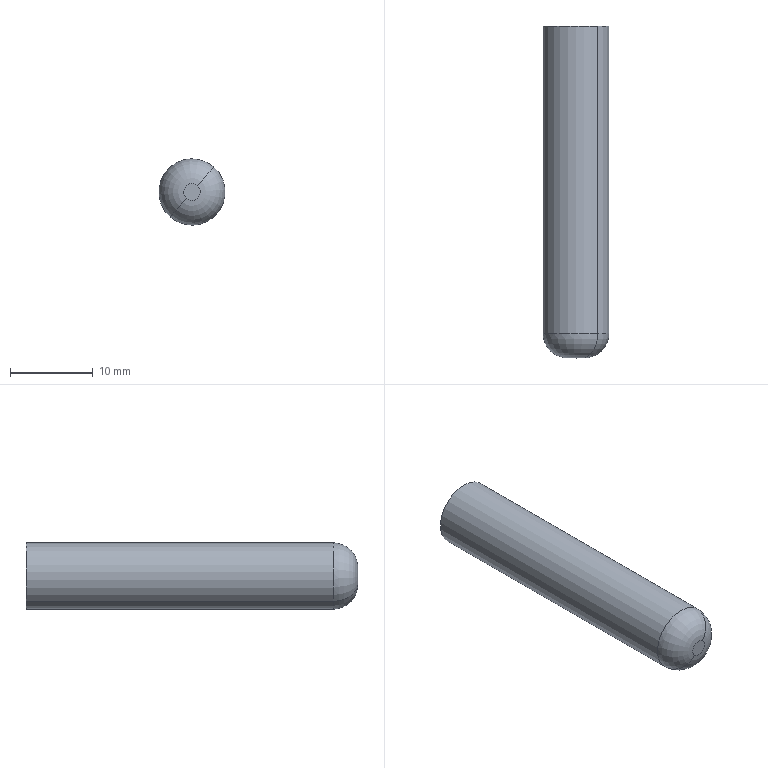Component | SolidWorks | NewDieSet-1_LocatingPin-1 | 1 solid | 6 faces | box 8 x 40 x 8 mm | volume 1970 mm3 | torus 2 | cylinder 2 | plane 2 | commonest cylinder face diameters 8 x2
build123d program:
from build123d import *

# Parameters (mm, degrees)
SKETCH1_R           = 4
BOSS_EXTRUDE1_DEPTH = 40
FILLET1_R           = 3


with BuildPart() as part:
    # Sketch1 → Boss-Extrude1 (new body)
    with BuildSketch(Plane.XY):
        Circle(SKETCH1_R)
    extrude(amount=BOSS_EXTRUDE1_DEPTH)

    # Fillet1
    fillet1_edges = [part.edges().sort_by_distance(p)[0] for p in [
        (-4, 0, 0),
    ]]
    fillet(fillet1_edges, radius=FILLET1_R)


solid = part.part

# Placed as in the assembly
solid = solid.moved(Location((-146.746, -9.073, 551.1), (-90, 0, 0)))
STEP:
#1=CARTESIAN_POINT('',(-5.803,-0.3572,21.667));
#2=VERTEX_POINT('',#1);
#3=CARTESIAN_POINT('',(-5.752,-0.3572,21.727));
#4=VERTEX_POINT('',#3);
#5=CARTESIAN_POINT('',(-5.777,-0.3572,21.697));
#6=DIRECTION('',(-0.,-1.,0.));
#7=DIRECTION('',(0.6544,0.,0.7562));
#8=AXIS2_PLACEMENT_3D('',#5,#6,#7);
#9=CIRCLE('',#8,0.03937);
#10=EDGE_CURVE('',#2,#4,#9,.T.);
#11=ORIENTED_EDGE('',*,*,#10,.F.);
#12=CARTESIAN_POINT('',(-5.88,-0.2391,21.578));
#13=VERTEX_POINT('',#12);
#14=CARTESIAN_POINT('',(-5.803,-0.2391,21.667));
#15=DIRECTION('',(0.7562,-0.,-0.6544));
#16=DIRECTION('',(-0.6544,0.,-0.7562));
#17=AXIS2_PLACEMENT_3D('',#14,#15,#16);
#18=CIRCLE('',#17,0.1181);
#19=EDGE_CURVE('',#2,#13,#18,.T.);
#20=ORIENTED_EDGE('',*,*,#19,.T.);
#21=CARTESIAN_POINT('',(-5.674,-0.2391,21.816));
#22=VERTEX_POINT('',#21);
#23=CARTESIAN_POINT('',(-5.777,-0.2391,21.697));
#24=DIRECTION('',(0.,1.,-0.));
#25=DIRECTION('',(0.6544,0.,0.7562));
#26=AXIS2_PLACEMENT_3D('',#23,#24,#25);
#27=CIRCLE('',#26,0.1575);
#28=EDGE_CURVE('',#22,#13,#27,.T.);
#29=ORIENTED_EDGE('',*,*,#28,.F.);
#30=CARTESIAN_POINT('',(-5.752,-0.2391,21.727));
#31=DIRECTION('',(-0.7562,0.,0.6544));
#32=DIRECTION('',(0.6544,0.,0.7562));
#33=AXIS2_PLACEMENT_3D('',#30,#31,#32);
#34=CIRCLE('',#33,0.1181);
#35=EDGE_CURVE('',#4,#22,#34,.T.);
#36=ORIENTED_EDGE('',*,*,#35,.F.);
#37=EDGE_LOOP('',(#11,#20,#29,#36));
#38=FACE_OUTER_BOUND('',#37,.T.);
#39=CARTESIAN_POINT('',(-5.777,-0.2391,21.697));
#40=DIRECTION('',(0.,1.,-0.));
#41=DIRECTION('',(0.6544,-0.,0.7562));
#42=AXIS2_PLACEMENT_3D('',#39,#40,#41);
#43=TOROIDAL_SURFACE('',#42,0.03937,0.1181);
#44=ADVANCED_FACE('',(#38),#43,.T.);
#45=CARTESIAN_POINT('',(-5.674,1.218,21.816));
#46=VERTEX_POINT('',#45);
#47=CARTESIAN_POINT('',(-5.88,1.218,21.578));
#48=VERTEX_POINT('',#47);
#49=CARTESIAN_POINT('',(-5.777,1.218,21.697));
#50=DIRECTION('',(0.,1.,-0.));
#51=DIRECTION('',(0.6544,0.,0.7562));
#52=AXIS2_PLACEMENT_3D('',#49,#50,#51);
#53=CIRCLE('',#52,0.1575);
#54=EDGE_CURVE('',#46,#48,#53,.T.);
#55=ORIENTED_EDGE('',*,*,#54,.F.);
#56=CARTESIAN_POINT('',(-5.674,1.218,21.816));
#57=DIRECTION('',(-0.,-1.,0.));
#58=VECTOR('',#57,39.37);
#59=LINE('',#56,#58);
#60=EDGE_CURVE('',#46,#22,#59,.T.);
#61=ORIENTED_EDGE('',*,*,#60,.T.);
#62=ORIENTED_EDGE('',*,*,#28,.T.);
#63=CARTESIAN_POINT('',(-5.88,1.218,21.578));
#64=DIRECTION('',(-0.,-1.,0.));
#65=VECTOR('',#64,39.37);
#66=LINE('',#63,#65);
#67=EDGE_CURVE('',#48,#13,#66,.T.);
#68=ORIENTED_EDGE('',*,*,#67,.F.);
#69=EDGE_LOOP('',(#55,#61,#62,#68));
#70=FACE_OUTER_BOUND('',#69,.T.);
#71=CARTESIAN_POINT('',(-5.777,1.218,21.697));
#72=DIRECTION('',(-0.,-1.,0.));
#73=DIRECTION('',(-0.6544,0.,-0.7562));
#74=AXIS2_PLACEMENT_3D('',#71,#72,#73);
#75=CYLINDRICAL_SURFACE('',#74,0.1575);
#76=ADVANCED_FACE('',(#70),#75,.T.);
#77=ORIENTED_EDGE('',*,*,#60,.F.);
#78=CARTESIAN_POINT('',(-5.777,1.218,21.697));
#79=DIRECTION('',(0.,1.,-0.));
#80=DIRECTION('',(0.6544,0.,0.7562));
#81=AXIS2_PLACEMENT_3D('',#78,#79,#80);
#82=CIRCLE('',#81,0.1575);
#83=EDGE_CURVE('',#48,#46,#82,.T.);
#84=ORIENTED_EDGE('',*,*,#83,.F.);
#85=ORIENTED_EDGE('',*,*,#67,.T.);
#86=CARTESIAN_POINT('',(-5.777,-0.2391,21.697));
#87=DIRECTION('',(0.,1.,-0.));
#88=DIRECTION('',(0.6544,0.,0.7562));
#89=AXIS2_PLACEMENT_3D('',#86,#87,#88);
#90=CIRCLE('',#89,0.1575);
#91=EDGE_CURVE('',#13,#22,#90,.T.);
#92=ORIENTED_EDGE('',*,*,#91,.T.);
#93=EDGE_LOOP('',(#77,#84,#85,#92));
#94=FACE_OUTER_BOUND('',#93,.T.);
#95=CARTESIAN_POINT('',(-5.777,1.218,21.697));
#96=DIRECTION('',(-0.,-1.,0.));
#97=DIRECTION('',(-0.6544,0.,-0.7562));
#98=AXIS2_PLACEMENT_3D('',#95,#96,#97);
#99=CYLINDRICAL_SURFACE('',#98,0.1575);
#100=ADVANCED_FACE('',(#94),#99,.T.);
#101=ORIENTED_EDGE('',*,*,#83,.T.);
#102=ORIENTED_EDGE('',*,*,#54,.T.);
#103=EDGE_LOOP('',(#101,#102));
#104=FACE_OUTER_BOUND('',#103,.T.);
#105=CARTESIAN_POINT('',(-5.777,1.218,21.697));
#106=DIRECTION('',(0.,1.,-0.));
#107=DIRECTION('',(0.6544,-0.,0.7562));
#108=AXIS2_PLACEMENT_3D('',#105,#106,#107);
#109=PLANE('',#108);
#110=ADVANCED_FACE('',(#104),#109,.T.);
#111=CARTESIAN_POINT('',(-5.777,-0.3572,21.697));
#112=DIRECTION('',(-0.,-1.,0.));
#113=DIRECTION('',(0.6544,0.,0.7562));
#114=AXIS2_PLACEMENT_3D('',#111,#112,#113);
#115=CIRCLE('',#114,0.03937);
#116=EDGE_CURVE('',#4,#2,#115,.T.);
#117=ORIENTED_EDGE('',*,*,#116,.T.);
#118=ORIENTED_EDGE('',*,*,#10,.T.);
#119=EDGE_LOOP('',(#117,#118));
#120=FACE_OUTER_BOUND('',#119,.T.);
#121=CARTESIAN_POINT('',(-5.777,-0.3572,21.697));
#122=DIRECTION('',(0.,1.,-0.));
#123=DIRECTION('',(0.6544,-0.,0.7562));
#124=AXIS2_PLACEMENT_3D('',#121,#122,#123);
#125=PLANE('',#124);
#126=ADVANCED_FACE('',(#120),#125,.F.);
#127=ORIENTED_EDGE('',*,*,#19,.F.);
#128=ORIENTED_EDGE('',*,*,#116,.F.);
#129=ORIENTED_EDGE('',*,*,#35,.T.);
#130=ORIENTED_EDGE('',*,*,#91,.F.);
#131=EDGE_LOOP('',(#127,#128,#129,#130));
#132=FACE_OUTER_BOUND('',#131,.T.);
#133=CARTESIAN_POINT('',(-5.777,-0.2391,21.697));
#134=DIRECTION('',(0.,1.,-0.));
#135=DIRECTION('',(0.6544,-0.,0.7562));
#136=AXIS2_PLACEMENT_3D('',#133,#134,#135);
#137=TOROIDAL_SURFACE('',#136,0.03937,0.1181);
#138=ADVANCED_FACE('',(#132),#137,.T.);
#139=CLOSED_SHELL('',(#44,#76,#100,#110,#126,#138));
#140=MANIFOLD_SOLID_BREP('',#139);
#141=CARTESIAN_POINT('',(0.,0.,0.));
#142=DIRECTION('',(0.,0.,1.));
#143=DIRECTION('',(1.,0.,0.));
#144=AXIS2_PLACEMENT_3D('',#141,#142,#143);
#145=(LENGTH_UNIT()NAMED_UNIT(*)SI_UNIT($,.METRE.));
#146=LENGTH_MEASURE_WITH_UNIT(LENGTH_MEASURE(0.0254),#145);
#147=DIMENSIONAL_EXPONENTS(1.,0.,0.,0.,0.,0.,0.);
#148=(CONVERSION_BASED_UNIT('',#146)LENGTH_UNIT()NAMED_UNIT(#147));
#149=UNCERTAINTY_MEASURE_WITH_UNIT(LENGTH_MEASURE(0.00001),#148,'','');
#150=(NAMED_UNIT(*)PLANE_ANGLE_UNIT()SI_UNIT($,.RADIAN.));
#151=(NAMED_UNIT(*)SI_UNIT($,.STERADIAN.)SOLID_ANGLE_UNIT());
#152=(GEOMETRIC_REPRESENTATION_CONTEXT(3)GLOBAL_UNCERTAINTY_ASSIGNED_CONTEXT((#149))GLOBAL_UNIT_ASSIGNED_CONTEXT((#148,#150,#151))REPRESENTATION_CONTEXT('',''));
#153=ADVANCED_BREP_SHAPE_REPRESENTATION('',(#140,#144),#152);
#154=COLOUR_RGB('',0.7922,0.8196,0.9333);
#155=FILL_AREA_STYLE_COLOUR('',#154);
#156=FILL_AREA_STYLE('',(#155));
#157=SURFACE_STYLE_FILL_AREA(#156);
#158=SURFACE_SIDE_STYLE('',(#157));
#159=SURFACE_STYLE_USAGE(.BOTH.,#158);
#160=PRESENTATION_STYLE_ASSIGNMENT((#159));
#161=STYLED_ITEM('',(#160),#140);
#162=(LENGTH_UNIT()NAMED_UNIT(*)SI_UNIT($,.METRE.));
#163=LENGTH_MEASURE_WITH_UNIT(LENGTH_MEASURE(0.0254),#162);
#164=DIMENSIONAL_EXPONENTS(1.,0.,0.,0.,0.,0.,0.);
#165=(CONVERSION_BASED_UNIT('',#163)LENGTH_UNIT()NAMED_UNIT(#164));
#166=UNCERTAINTY_MEASURE_WITH_UNIT(LENGTH_MEASURE(0.00001),#165,'','');
#167=(NAMED_UNIT(*)PLANE_ANGLE_UNIT()SI_UNIT($,.RADIAN.));
#168=(NAMED_UNIT(*)SI_UNIT($,.STERADIAN.)SOLID_ANGLE_UNIT());
#169=(GEOMETRIC_REPRESENTATION_CONTEXT(3)GLOBAL_UNCERTAINTY_ASSIGNED_CONTEXT((#166))GLOBAL_UNIT_ASSIGNED_CONTEXT((#165,#167,#168))REPRESENTATION_CONTEXT('',''));
#170=MECHANICAL_DESIGN_GEOMETRIC_PRESENTATION_REPRESENTATION('',(#161),#169);
#171=PRESENTATION_LAYER_ASSIGNMENT('','',(#161));